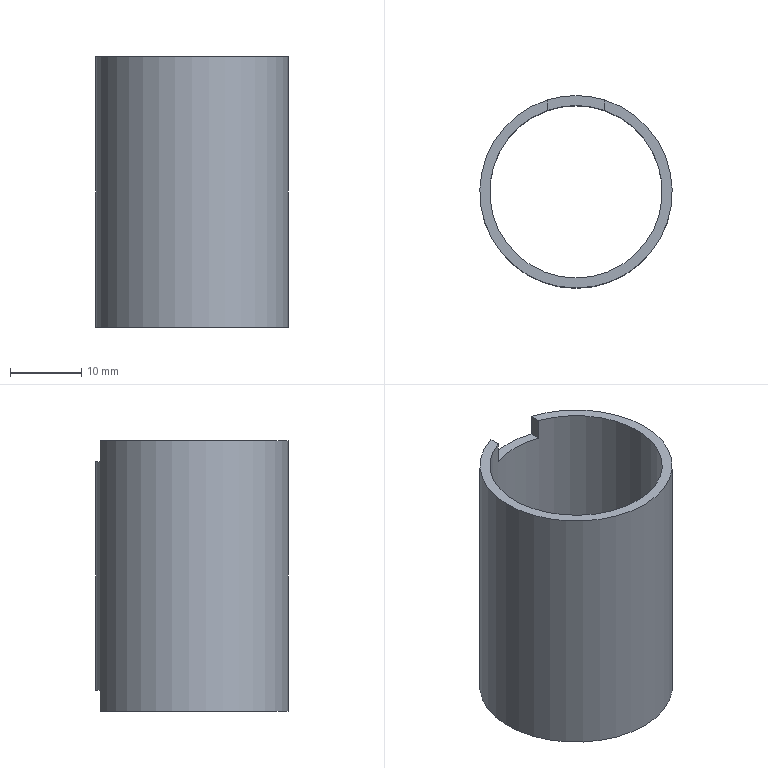Component | NX | UPPER_PISTON_CYLINDER_LINER | 1 solid | 10 faces | box 27 x 27 x 38 mm | volume 4210 mm3 | plane 8 | cylinder 2 | commonest cylinder face diameters 27 x1 24.2 x1
STEP:
#1=CARTESIAN_POINT('',(0.,0.,0.));
#2=DIRECTION('',(0.,0.,1.));
#3=DIRECTION('',(1.,0.,0.));
#4=AXIS2_PLACEMENT_3D('',#1,#2,#3);
#5=CARTESIAN_POINT('',(4.,2.894,162.5));
#6=VERTEX_POINT('',#5);
#7=CARTESIAN_POINT('',(4.,2.894,159.5));
#8=VERTEX_POINT('',#7);
#9=CARTESIAN_POINT('',(4.,2.894,162.5));
#10=DIRECTION('',(0.,0.,-1.));
#11=VECTOR('',#10,1.);
#12=LINE('',#9,#11);
#13=CARTESIAN_POINT('',(-0.,-10.,162.5));
#14=DIRECTION('',(0.,0.,-1.));
#15=DIRECTION('',(1.,0.,0.));
#16=AXIS2_PLACEMENT_3D('',#13,#14,#15);
#17=CYLINDRICAL_SURFACE('',#16,13.5);
#18=CARTESIAN_POINT('',(5.013,0.));
#19=DIRECTION('',(0.,1.));
#20=VECTOR('',#19,1.);
#21=LINE('',#18,#20);
#22=(GEOMETRIC_REPRESENTATION_CONTEXT(2)PARAMETRIC_REPRESENTATION_CONTEXT()REPRESENTATION_CONTEXT('',''));
#23=DEFINITIONAL_REPRESENTATION('',(#21),#22);
#24=PCURVE('',#17,#23);
#25=CARTESIAN_POINT('',(4.,-3.333,159.5));
#26=DIRECTION('',(1.,0.,0.));
#27=DIRECTION('',(0.,0.,1.));
#28=AXIS2_PLACEMENT_3D('',#25,#26,#27);
#29=PLANE('',#28);
#30=CARTESIAN_POINT('',(3.,-6.227));
#31=DIRECTION('',(-1.,0.));
#32=VECTOR('',#31,1.);
#33=LINE('',#30,#32);
#34=(GEOMETRIC_REPRESENTATION_CONTEXT(2)PARAMETRIC_REPRESENTATION_CONTEXT()REPRESENTATION_CONTEXT('',''));
#35=DEFINITIONAL_REPRESENTATION('',(#33),#34);
#36=PCURVE('',#29,#35);
#37=SURFACE_CURVE('',#12,(#24,#36),.PCURVE_S1.);
#38=EDGE_CURVE('',#6,#8,#37,.T.);
#39=ORIENTED_EDGE('',*,*,#38,.F.);
#40=CARTESIAN_POINT('',(-4.,2.894,162.5));
#41=VERTEX_POINT('',#40);
#42=CARTESIAN_POINT('',(-0.,-10.,162.5));
#43=DIRECTION('',(0.,0.,-1.));
#44=DIRECTION('',(-1.,-0.,0.));
#45=AXIS2_PLACEMENT_3D('',#42,#43,#44);
#46=CIRCLE('',#45,13.5);
#47=CARTESIAN_POINT('',(3.142,0.));
#48=DIRECTION('',(1.,0.));
#49=VECTOR('',#48,1.);
#50=LINE('',#47,#49);
#51=(GEOMETRIC_REPRESENTATION_CONTEXT(2)PARAMETRIC_REPRESENTATION_CONTEXT()REPRESENTATION_CONTEXT('',''));
#52=DEFINITIONAL_REPRESENTATION('',(#50),#51);
#53=PCURVE('',#17,#52);
#54=CARTESIAN_POINT('',(-0.,-10.,162.5));
#55=DIRECTION('',(0.,0.,-1.));
#56=DIRECTION('',(1.,0.,0.));
#57=AXIS2_PLACEMENT_3D('',#54,#55,#56);
#58=PLANE('',#57);
#59=CARTESIAN_POINT('',(0.,0.));
#60=DIRECTION('',(-1.,0.));
#61=AXIS2_PLACEMENT_2D('',#59,#60);
#62=CIRCLE('',#61,13.5);
#63=(GEOMETRIC_REPRESENTATION_CONTEXT(2)PARAMETRIC_REPRESENTATION_CONTEXT()REPRESENTATION_CONTEXT('',''));
#64=DEFINITIONAL_REPRESENTATION('',(#62),#63);
#65=PCURVE('',#58,#64);
#66=SURFACE_CURVE('',#46,(#53,#65),.PCURVE_S1.);
#67=EDGE_CURVE('',#6,#41,#66,.T.);
#68=ORIENTED_EDGE('',*,*,#67,.T.);
#69=CARTESIAN_POINT('',(-4.,2.894,159.5));
#70=VERTEX_POINT('',#69);
#71=CARTESIAN_POINT('',(-4.,2.894,162.5));
#72=DIRECTION('',(0.,0.,1.));
#73=VECTOR('',#72,1.);
#74=LINE('',#71,#73);
#75=CARTESIAN_POINT('',(10.695,0.));
#76=DIRECTION('',(0.,-1.));
#77=VECTOR('',#76,1.);
#78=LINE('',#75,#77);
#79=(GEOMETRIC_REPRESENTATION_CONTEXT(2)PARAMETRIC_REPRESENTATION_CONTEXT()REPRESENTATION_CONTEXT('',''));
#80=DEFINITIONAL_REPRESENTATION('',(#78),#79);
#81=PCURVE('',#17,#80);
#82=CARTESIAN_POINT('',(-4.,5.111,159.5));
#83=DIRECTION('',(-1.,0.,0.));
#84=DIRECTION('',(-0.,-1.,0.));
#85=AXIS2_PLACEMENT_3D('',#82,#83,#84);
#86=PLANE('',#85);
#87=CARTESIAN_POINT('',(2.217,3.));
#88=DIRECTION('',(0.,1.));
#89=VECTOR('',#88,1.);
#90=LINE('',#87,#89);
#91=(GEOMETRIC_REPRESENTATION_CONTEXT(2)PARAMETRIC_REPRESENTATION_CONTEXT()REPRESENTATION_CONTEXT('',''));
#92=DEFINITIONAL_REPRESENTATION('',(#90),#91);
#93=PCURVE('',#86,#92);
#94=SURFACE_CURVE('',#74,(#81,#93),.PCURVE_S1.);
#95=EDGE_CURVE('',#70,#41,#94,.T.);
#96=ORIENTED_EDGE('',*,*,#95,.F.);
#97=CARTESIAN_POINT('',(-0.,-10.,159.5));
#98=DIRECTION('',(0.,0.,-1.));
#99=DIRECTION('',(-1.,0.,0.));
#100=AXIS2_PLACEMENT_3D('',#97,#98,#99);
#101=CIRCLE('',#100,13.5);
#102=CARTESIAN_POINT('',(9.425,3.));
#103=DIRECTION('',(1.,0.));
#104=VECTOR('',#103,1.);
#105=LINE('',#102,#104);
#106=(GEOMETRIC_REPRESENTATION_CONTEXT(2)PARAMETRIC_REPRESENTATION_CONTEXT()REPRESENTATION_CONTEXT('',''));
#107=DEFINITIONAL_REPRESENTATION('',(#105),#106);
#108=PCURVE('',#17,#107);
#109=CARTESIAN_POINT('',(-0.,-10.,159.5));
#110=DIRECTION('',(0.,0.,1.));
#111=DIRECTION('',(-1.,0.,0.));
#112=AXIS2_PLACEMENT_3D('',#109,#110,#111);
#113=PLANE('',#112);
#114=CARTESIAN_POINT('',(13.5,0.));
#115=CARTESIAN_POINT('',(13.5,-23.383));
#116=CARTESIAN_POINT('',(-6.75,-11.691));
#117=CARTESIAN_POINT('',(-27.,-0.));
#118=CARTESIAN_POINT('',(-6.75,11.691));
#119=CARTESIAN_POINT('',(13.5,23.383));
#120=CARTESIAN_POINT('',(13.5,0.));
#121=(BOUNDED_CURVE()B_SPLINE_CURVE(2,(#114,#115,#116,#117,#118,#119,#120),.UNSPECIFIED.,.T.,.F.)B_SPLINE_CURVE_WITH_KNOTS((1,2,2,2,2,1),(-2.094,0.,2.094,4.189,6.283,8.378),.UNSPECIFIED.)CURVE()GEOMETRIC_REPRESENTATION_ITEM()RATIONAL_B_SPLINE_CURVE((1.,0.5,1.,0.5,1.,0.5,1.))REPRESENTATION_ITEM(''));
#122=(GEOMETRIC_REPRESENTATION_CONTEXT(2)PARAMETRIC_REPRESENTATION_CONTEXT()REPRESENTATION_CONTEXT('',''));
#123=DEFINITIONAL_REPRESENTATION('',(#121),#122);
#124=PCURVE('',#113,#123);
#125=SURFACE_CURVE('',#101,(#108,#124),.PCURVE_S1.);
#126=EDGE_CURVE('',#70,#8,#125,.T.);
#127=ORIENTED_EDGE('',*,*,#126,.T.);
#128=CARTESIAN_POINT('',(4.,2.894,127.5));
#129=VERTEX_POINT('',#128);
#130=CARTESIAN_POINT('',(4.,2.894,159.5));
#131=CARTESIAN_POINT('',(4.,2.894,127.5));
#132=B_SPLINE_CURVE_WITH_KNOTS('',1,(#130,#131),.UNSPECIFIED.,.F.,.F.,(2,2),(3.,35.),.PIECEWISE_BEZIER_KNOTS.);
#133=CARTESIAN_POINT('',(11.296,0.));
#134=DIRECTION('',(0.,1.));
#135=VECTOR('',#134,1.);
#136=LINE('',#133,#135);
#137=(GEOMETRIC_REPRESENTATION_CONTEXT(2)PARAMETRIC_REPRESENTATION_CONTEXT()REPRESENTATION_CONTEXT('',''));
#138=DEFINITIONAL_REPRESENTATION('',(#136),#137);
#139=PCURVE('',#17,#138);
#140=CARTESIAN_POINT('',(5.013,0.));
#141=DIRECTION('',(0.,1.));
#142=VECTOR('',#141,1.);
#143=LINE('',#140,#142);
#144=(GEOMETRIC_REPRESENTATION_CONTEXT(2)PARAMETRIC_REPRESENTATION_CONTEXT()REPRESENTATION_CONTEXT('',''));
#145=DEFINITIONAL_REPRESENTATION('',(#143),#144);
#146=PCURVE('',#17,#145);
#147=SEAM_CURVE('',#132,(#139,#146),.PCURVE_S1.);
#148=EDGE_CURVE('',#8,#129,#147,.T.);
#149=ORIENTED_EDGE('',*,*,#148,.T.);
#150=CARTESIAN_POINT('',(-4.,2.894,127.5));
#151=VERTEX_POINT('',#150);
#152=CARTESIAN_POINT('',(-0.,-10.,127.5));
#153=DIRECTION('',(0.,0.,-1.));
#154=DIRECTION('',(-1.,0.,0.));
#155=AXIS2_PLACEMENT_3D('',#152,#153,#154);
#156=CIRCLE('',#155,13.5);
#157=CARTESIAN_POINT('',(9.425,35.));
#158=DIRECTION('',(1.,0.));
#159=VECTOR('',#158,1.);
#160=LINE('',#157,#159);
#161=(GEOMETRIC_REPRESENTATION_CONTEXT(2)PARAMETRIC_REPRESENTATION_CONTEXT()REPRESENTATION_CONTEXT('',''));
#162=DEFINITIONAL_REPRESENTATION('',(#160),#161);
#163=PCURVE('',#17,#162);
#164=CARTESIAN_POINT('',(-0.,-10.,127.5));
#165=DIRECTION('',(0.,0.,1.));
#166=DIRECTION('',(-1.,0.,0.));
#167=AXIS2_PLACEMENT_3D('',#164,#165,#166);
#168=PLANE('',#167);
#169=CARTESIAN_POINT('',(13.5,0.));
#170=CARTESIAN_POINT('',(13.5,-23.383));
#171=CARTESIAN_POINT('',(-6.75,-11.691));
#172=CARTESIAN_POINT('',(-27.,-0.));
#173=CARTESIAN_POINT('',(-6.75,11.691));
#174=CARTESIAN_POINT('',(13.5,23.383));
#175=CARTESIAN_POINT('',(13.5,0.));
#176=(BOUNDED_CURVE()B_SPLINE_CURVE(2,(#169,#170,#171,#172,#173,#174,#175),.UNSPECIFIED.,.T.,.F.)B_SPLINE_CURVE_WITH_KNOTS((1,2,2,2,2,1),(-2.094,0.,2.094,4.189,6.283,8.378),.UNSPECIFIED.)CURVE()GEOMETRIC_REPRESENTATION_ITEM()RATIONAL_B_SPLINE_CURVE((1.,0.5,1.,0.5,1.,0.5,1.))REPRESENTATION_ITEM(''));
#177=(GEOMETRIC_REPRESENTATION_CONTEXT(2)PARAMETRIC_REPRESENTATION_CONTEXT()REPRESENTATION_CONTEXT('',''));
#178=DEFINITIONAL_REPRESENTATION('',(#176),#177);
#179=PCURVE('',#168,#178);
#180=SURFACE_CURVE('',#156,(#163,#179),.PCURVE_S1.);
#181=EDGE_CURVE('',#151,#129,#180,.T.);
#182=ORIENTED_EDGE('',*,*,#181,.F.);
#183=CARTESIAN_POINT('',(-4.,2.894,124.5));
#184=VERTEX_POINT('',#183);
#185=CARTESIAN_POINT('',(-4.,2.894,162.5));
#186=DIRECTION('',(0.,0.,-1.));
#187=VECTOR('',#186,1.);
#188=LINE('',#185,#187);
#189=CARTESIAN_POINT('',(10.695,0.));
#190=DIRECTION('',(0.,1.));
#191=VECTOR('',#190,1.);
#192=LINE('',#189,#191);
#193=(GEOMETRIC_REPRESENTATION_CONTEXT(2)PARAMETRIC_REPRESENTATION_CONTEXT()REPRESENTATION_CONTEXT('',''));
#194=DEFINITIONAL_REPRESENTATION('',(#192),#193);
#195=PCURVE('',#17,#194);
#196=CARTESIAN_POINT('',(-4.,5.111,127.5));
#197=DIRECTION('',(1.,-0.,0.));
#198=DIRECTION('',(0.,1.,0.));
#199=AXIS2_PLACEMENT_3D('',#196,#197,#198);
#200=PLANE('',#199);
#201=CARTESIAN_POINT('',(-2.217,35.));
#202=DIRECTION('',(0.,-1.));
#203=VECTOR('',#202,1.);
#204=LINE('',#201,#203);
#205=(GEOMETRIC_REPRESENTATION_CONTEXT(2)PARAMETRIC_REPRESENTATION_CONTEXT()REPRESENTATION_CONTEXT('',''));
#206=DEFINITIONAL_REPRESENTATION('',(#204),#205);
#207=PCURVE('',#200,#206);
#208=SURFACE_CURVE('',#188,(#195,#207),.PCURVE_S1.);
#209=EDGE_CURVE('',#151,#184,#208,.T.);
#210=ORIENTED_EDGE('',*,*,#209,.T.);
#211=CARTESIAN_POINT('',(4.,2.894,124.5));
#212=VERTEX_POINT('',#211);
#213=CARTESIAN_POINT('',(-0.,-10.,124.5));
#214=DIRECTION('',(0.,0.,-1.));
#215=DIRECTION('',(-1.,-0.,0.));
#216=AXIS2_PLACEMENT_3D('',#213,#214,#215);
#217=CIRCLE('',#216,13.5);
#218=CARTESIAN_POINT('',(3.142,38.));
#219=DIRECTION('',(1.,0.));
#220=VECTOR('',#219,1.);
#221=LINE('',#218,#220);
#222=(GEOMETRIC_REPRESENTATION_CONTEXT(2)PARAMETRIC_REPRESENTATION_CONTEXT()REPRESENTATION_CONTEXT('',''));
#223=DEFINITIONAL_REPRESENTATION('',(#221),#222);
#224=PCURVE('',#17,#223);
#225=CARTESIAN_POINT('',(-0.,-10.,124.5));
#226=DIRECTION('',(0.,0.,-1.));
#227=DIRECTION('',(1.,0.,0.));
#228=AXIS2_PLACEMENT_3D('',#225,#226,#227);
#229=PLANE('',#228);
#230=CARTESIAN_POINT('',(0.,0.));
#231=DIRECTION('',(-1.,0.));
#232=AXIS2_PLACEMENT_2D('',#230,#231);
#233=CIRCLE('',#232,13.5);
#234=(GEOMETRIC_REPRESENTATION_CONTEXT(2)PARAMETRIC_REPRESENTATION_CONTEXT()REPRESENTATION_CONTEXT('',''));
#235=DEFINITIONAL_REPRESENTATION('',(#233),#234);
#236=PCURVE('',#229,#235);
#237=SURFACE_CURVE('',#217,(#224,#236),.PCURVE_S1.);
#238=EDGE_CURVE('',#212,#184,#237,.T.);
#239=ORIENTED_EDGE('',*,*,#238,.F.);
#240=CARTESIAN_POINT('',(4.,2.894,162.5));
#241=DIRECTION('',(0.,0.,1.));
#242=VECTOR('',#241,1.);
#243=LINE('',#240,#242);
#244=CARTESIAN_POINT('',(5.013,0.));
#245=DIRECTION('',(0.,-1.));
#246=VECTOR('',#245,1.);
#247=LINE('',#244,#246);
#248=(GEOMETRIC_REPRESENTATION_CONTEXT(2)PARAMETRIC_REPRESENTATION_CONTEXT()REPRESENTATION_CONTEXT('',''));
#249=DEFINITIONAL_REPRESENTATION('',(#247),#248);
#250=PCURVE('',#17,#249);
#251=CARTESIAN_POINT('',(4.,-3.333,127.5));
#252=DIRECTION('',(-1.,0.,0.));
#253=DIRECTION('',(0.,0.,-1.));
#254=AXIS2_PLACEMENT_3D('',#251,#252,#253);
#255=PLANE('',#254);
#256=CARTESIAN_POINT('',(-35.,-6.227));
#257=DIRECTION('',(-1.,0.));
#258=VECTOR('',#257,1.);
#259=LINE('',#256,#258);
#260=(GEOMETRIC_REPRESENTATION_CONTEXT(2)PARAMETRIC_REPRESENTATION_CONTEXT()REPRESENTATION_CONTEXT('',''));
#261=DEFINITIONAL_REPRESENTATION('',(#259),#260);
#262=PCURVE('',#255,#261);
#263=SURFACE_CURVE('',#243,(#250,#262),.PCURVE_S1.);
#264=EDGE_CURVE('',#212,#129,#263,.T.);
#265=ORIENTED_EDGE('',*,*,#264,.T.);
#266=ORIENTED_EDGE('',*,*,#148,.F.);
#267=EDGE_LOOP('',(#39,#68,#96,#127,#149,#182,#210,#239,#265,#266));
#268=FACE_BOUND('',#267,.T.);
#269=ADVANCED_FACE('',(#268),#17,.T.);
#270=CARTESIAN_POINT('',(4.,1.42,124.5));
#271=VERTEX_POINT('',#270);
#272=CARTESIAN_POINT('',(-4.,1.42,124.5));
#273=VERTEX_POINT('',#272);
#274=CARTESIAN_POINT('',(0.,-10.,124.5));
#275=DIRECTION('',(0.,0.,-1.));
#276=DIRECTION('',(1.,0.,0.));
#277=AXIS2_PLACEMENT_3D('',#274,#275,#276);
#278=CIRCLE('',#277,12.1);
#279=CARTESIAN_POINT('',(0.,0.));
#280=DIRECTION('',(1.,0.));
#281=AXIS2_PLACEMENT_2D('',#279,#280);
#282=CIRCLE('',#281,12.1);
#283=(GEOMETRIC_REPRESENTATION_CONTEXT(2)PARAMETRIC_REPRESENTATION_CONTEXT()REPRESENTATION_CONTEXT('',''));
#284=DEFINITIONAL_REPRESENTATION('',(#282),#283);
#285=PCURVE('',#229,#284);
#286=CARTESIAN_POINT('',(0.,-10.,124.4));
#287=DIRECTION('',(0.,0.,1.));
#288=DIRECTION('',(-1.,0.,0.));
#289=AXIS2_PLACEMENT_3D('',#286,#287,#288);
#290=CYLINDRICAL_SURFACE('',#289,12.1);
#291=CARTESIAN_POINT('',(15.708,0.1));
#292=DIRECTION('',(-1.,0.));
#293=VECTOR('',#292,1.);
#294=LINE('',#291,#293);
#295=(GEOMETRIC_REPRESENTATION_CONTEXT(2)PARAMETRIC_REPRESENTATION_CONTEXT()REPRESENTATION_CONTEXT('',''));
#296=DEFINITIONAL_REPRESENTATION('',(#294),#295);
#297=PCURVE('',#290,#296);
#298=SURFACE_CURVE('',#278,(#285,#297),.PCURVE_S1.);
#299=EDGE_CURVE('',#271,#273,#298,.T.);
#300=ORIENTED_EDGE('',*,*,#299,.F.);
#301=CARTESIAN_POINT('',(4.,-3.333,124.5));
#302=DIRECTION('',(0.,1.,0.));
#303=VECTOR('',#302,1.);
#304=LINE('',#301,#303);
#305=CARTESIAN_POINT('',(4.,-6.667));
#306=DIRECTION('',(0.,-1.));
#307=VECTOR('',#306,1.);
#308=LINE('',#305,#307);
#309=(GEOMETRIC_REPRESENTATION_CONTEXT(2)PARAMETRIC_REPRESENTATION_CONTEXT()REPRESENTATION_CONTEXT('',''));
#310=DEFINITIONAL_REPRESENTATION('',(#308),#309);
#311=PCURVE('',#229,#310);
#312=CARTESIAN_POINT('',(3.,0.));
#313=DIRECTION('',(0.,-1.));
#314=VECTOR('',#313,1.);
#315=LINE('',#312,#314);
#316=(GEOMETRIC_REPRESENTATION_CONTEXT(2)PARAMETRIC_REPRESENTATION_CONTEXT()REPRESENTATION_CONTEXT('',''));
#317=DEFINITIONAL_REPRESENTATION('',(#315),#316);
#318=PCURVE('',#255,#317);
#319=SURFACE_CURVE('',#304,(#311,#318),.PCURVE_S1.);
#320=EDGE_CURVE('',#271,#212,#319,.T.);
#321=ORIENTED_EDGE('',*,*,#320,.T.);
#322=ORIENTED_EDGE('',*,*,#238,.T.);
#323=CARTESIAN_POINT('',(-4.,5.111,124.5));
#324=DIRECTION('',(-0.,-1.,0.));
#325=VECTOR('',#324,1.);
#326=LINE('',#323,#325);
#327=CARTESIAN_POINT('',(-4.,-15.111));
#328=DIRECTION('',(-0.,1.));
#329=VECTOR('',#328,1.);
#330=LINE('',#327,#329);
#331=(GEOMETRIC_REPRESENTATION_CONTEXT(2)PARAMETRIC_REPRESENTATION_CONTEXT()REPRESENTATION_CONTEXT('',''));
#332=DEFINITIONAL_REPRESENTATION('',(#330),#331);
#333=PCURVE('',#229,#332);
#334=CARTESIAN_POINT('',(0.,-3.));
#335=DIRECTION('',(-1.,0.));
#336=VECTOR('',#335,1.);
#337=LINE('',#334,#336);
#338=(GEOMETRIC_REPRESENTATION_CONTEXT(2)PARAMETRIC_REPRESENTATION_CONTEXT()REPRESENTATION_CONTEXT('',''));
#339=DEFINITIONAL_REPRESENTATION('',(#337),#338);
#340=PCURVE('',#200,#339);
#341=SURFACE_CURVE('',#326,(#333,#340),.PCURVE_S1.);
#342=EDGE_CURVE('',#184,#273,#341,.T.);
#343=ORIENTED_EDGE('',*,*,#342,.T.);
#344=EDGE_LOOP('',(#300,#321,#322,#343));
#345=FACE_BOUND('',#344,.T.);
#346=ADVANCED_FACE('',(#345),#229,.T.);
#347=CARTESIAN_POINT('',(4.,1.42,162.5));
#348=VERTEX_POINT('',#347);
#349=CARTESIAN_POINT('',(4.,-3.333,162.5));
#350=DIRECTION('',(0.,1.,0.));
#351=VECTOR('',#350,1.);
#352=LINE('',#349,#351);
#353=CARTESIAN_POINT('',(4.,-6.667));
#354=DIRECTION('',(0.,-1.));
#355=VECTOR('',#354,1.);
#356=LINE('',#353,#355);
#357=(GEOMETRIC_REPRESENTATION_CONTEXT(2)PARAMETRIC_REPRESENTATION_CONTEXT()REPRESENTATION_CONTEXT('',''));
#358=DEFINITIONAL_REPRESENTATION('',(#356),#357);
#359=PCURVE('',#58,#358);
#360=CARTESIAN_POINT('',(3.,0.));
#361=DIRECTION('',(0.,-1.));
#362=VECTOR('',#361,1.);
#363=LINE('',#360,#362);
#364=(GEOMETRIC_REPRESENTATION_CONTEXT(2)PARAMETRIC_REPRESENTATION_CONTEXT()REPRESENTATION_CONTEXT('',''));
#365=DEFINITIONAL_REPRESENTATION('',(#363),#364);
#366=PCURVE('',#29,#365);
#367=SURFACE_CURVE('',#352,(#359,#366),.PCURVE_S1.);
#368=EDGE_CURVE('',#348,#6,#367,.T.);
#369=ORIENTED_EDGE('',*,*,#368,.F.);
#370=CARTESIAN_POINT('',(-4.,1.42,162.5));
#371=VERTEX_POINT('',#370);
#372=CARTESIAN_POINT('',(0.,-10.,162.5));
#373=DIRECTION('',(0.,0.,-1.));
#374=DIRECTION('',(1.,0.,0.));
#375=AXIS2_PLACEMENT_3D('',#372,#373,#374);
#376=CIRCLE('',#375,12.1);
#377=CARTESIAN_POINT('',(0.,0.));
#378=DIRECTION('',(1.,0.));
#379=AXIS2_PLACEMENT_2D('',#377,#378);
#380=CIRCLE('',#379,12.1);
#381=(GEOMETRIC_REPRESENTATION_CONTEXT(2)PARAMETRIC_REPRESENTATION_CONTEXT()REPRESENTATION_CONTEXT('',''));
#382=DEFINITIONAL_REPRESENTATION('',(#380),#381);
#383=PCURVE('',#58,#382);
#384=CARTESIAN_POINT('',(15.708,38.1));
#385=DIRECTION('',(-1.,0.));
#386=VECTOR('',#385,1.);
#387=LINE('',#384,#386);
#388=(GEOMETRIC_REPRESENTATION_CONTEXT(2)PARAMETRIC_REPRESENTATION_CONTEXT()REPRESENTATION_CONTEXT('',''));
#389=DEFINITIONAL_REPRESENTATION('',(#387),#388);
#390=PCURVE('',#290,#389);
#391=SURFACE_CURVE('',#376,(#383,#390),.PCURVE_S1.);
#392=EDGE_CURVE('',#348,#371,#391,.T.);
#393=ORIENTED_EDGE('',*,*,#392,.T.);
#394=CARTESIAN_POINT('',(-4.,5.111,162.5));
#395=DIRECTION('',(-0.,-1.,0.));
#396=VECTOR('',#395,1.);
#397=LINE('',#394,#396);
#398=CARTESIAN_POINT('',(-4.,-15.111));
#399=DIRECTION('',(-0.,1.));
#400=VECTOR('',#399,1.);
#401=LINE('',#398,#400);
#402=(GEOMETRIC_REPRESENTATION_CONTEXT(2)PARAMETRIC_REPRESENTATION_CONTEXT()REPRESENTATION_CONTEXT('',''));
#403=DEFINITIONAL_REPRESENTATION('',(#401),#402);
#404=PCURVE('',#58,#403);
#405=CARTESIAN_POINT('',(0.,3.));
#406=DIRECTION('',(1.,0.));
#407=VECTOR('',#406,1.);
#408=LINE('',#405,#407);
#409=(GEOMETRIC_REPRESENTATION_CONTEXT(2)PARAMETRIC_REPRESENTATION_CONTEXT()REPRESENTATION_CONTEXT('',''));
#410=DEFINITIONAL_REPRESENTATION('',(#408),#409);
#411=PCURVE('',#86,#410);
#412=SURFACE_CURVE('',#397,(#404,#411),.PCURVE_S1.);
#413=EDGE_CURVE('',#41,#371,#412,.T.);
#414=ORIENTED_EDGE('',*,*,#413,.F.);
#415=ORIENTED_EDGE('',*,*,#67,.F.);
#416=EDGE_LOOP('',(#369,#393,#414,#415));
#417=FACE_BOUND('',#416,.T.);
#418=ADVANCED_FACE('',(#417),#58,.F.);
#419=CARTESIAN_POINT('',(4.,1.42,159.5));
#420=VERTEX_POINT('',#419);
#421=CARTESIAN_POINT('',(-4.,1.42,159.5));
#422=VERTEX_POINT('',#421);
#423=CARTESIAN_POINT('',(0.,-10.,159.5));
#424=DIRECTION('',(0.,0.,1.));
#425=DIRECTION('',(-1.,0.,0.));
#426=AXIS2_PLACEMENT_3D('',#423,#424,#425);
#427=CIRCLE('',#426,12.1);
#428=CARTESIAN_POINT('',(-0.,0.));
#429=DIRECTION('',(1.,0.));
#430=AXIS2_PLACEMENT_2D('',#428,#429);
#431=CIRCLE('',#430,12.1);
#432=(GEOMETRIC_REPRESENTATION_CONTEXT(2)PARAMETRIC_REPRESENTATION_CONTEXT()REPRESENTATION_CONTEXT('',''));
#433=DEFINITIONAL_REPRESENTATION('',(#431),#432);
#434=PCURVE('',#113,#433);
#435=CARTESIAN_POINT('',(6.283,35.1));
#436=DIRECTION('',(1.,0.));
#437=VECTOR('',#436,1.);
#438=LINE('',#435,#437);
#439=(GEOMETRIC_REPRESENTATION_CONTEXT(2)PARAMETRIC_REPRESENTATION_CONTEXT()REPRESENTATION_CONTEXT('',''));
#440=DEFINITIONAL_REPRESENTATION('',(#438),#439);
#441=PCURVE('',#290,#440);
#442=SURFACE_CURVE('',#427,(#434,#441),.PCURVE_S1.);
#443=EDGE_CURVE('',#420,#422,#442,.T.);
#444=ORIENTED_EDGE('',*,*,#443,.F.);
#445=CARTESIAN_POINT('',(4.,-3.333,159.5));
#446=DIRECTION('',(0.,-1.,0.));
#447=VECTOR('',#446,1.);
#448=LINE('',#445,#447);
#449=CARTESIAN_POINT('',(-4.,-6.667));
#450=DIRECTION('',(0.,1.));
#451=VECTOR('',#450,1.);
#452=LINE('',#449,#451);
#453=(GEOMETRIC_REPRESENTATION_CONTEXT(2)PARAMETRIC_REPRESENTATION_CONTEXT()REPRESENTATION_CONTEXT('',''));
#454=DEFINITIONAL_REPRESENTATION('',(#452),#453);
#455=PCURVE('',#113,#454);
#456=CARTESIAN_POINT('',(0.,0.));
#457=DIRECTION('',(0.,1.));
#458=VECTOR('',#457,1.);
#459=LINE('',#456,#458);
#460=(GEOMETRIC_REPRESENTATION_CONTEXT(2)PARAMETRIC_REPRESENTATION_CONTEXT()REPRESENTATION_CONTEXT('',''));
#461=DEFINITIONAL_REPRESENTATION('',(#459),#460);
#462=PCURVE('',#29,#461);
#463=SURFACE_CURVE('',#448,(#455,#462),.PCURVE_S1.);
#464=EDGE_CURVE('',#8,#420,#463,.T.);
#465=ORIENTED_EDGE('',*,*,#464,.F.);
#466=ORIENTED_EDGE('',*,*,#126,.F.);
#467=CARTESIAN_POINT('',(-4.,5.111,159.5));
#468=DIRECTION('',(0.,1.,0.));
#469=VECTOR('',#468,1.);
#470=LINE('',#467,#469);
#471=CARTESIAN_POINT('',(4.,-15.111));
#472=DIRECTION('',(-0.,-1.));
#473=VECTOR('',#472,1.);
#474=LINE('',#471,#473);
#475=(GEOMETRIC_REPRESENTATION_CONTEXT(2)PARAMETRIC_REPRESENTATION_CONTEXT()REPRESENTATION_CONTEXT('',''));
#476=DEFINITIONAL_REPRESENTATION('',(#474),#475);
#477=PCURVE('',#113,#476);
#478=CARTESIAN_POINT('',(0.,0.));
#479=DIRECTION('',(-1.,0.));
#480=VECTOR('',#479,1.);
#481=LINE('',#478,#480);
#482=(GEOMETRIC_REPRESENTATION_CONTEXT(2)PARAMETRIC_REPRESENTATION_CONTEXT()REPRESENTATION_CONTEXT('',''));
#483=DEFINITIONAL_REPRESENTATION('',(#481),#482);
#484=PCURVE('',#86,#483);
#485=SURFACE_CURVE('',#470,(#477,#484),.PCURVE_S1.);
#486=EDGE_CURVE('',#422,#70,#485,.T.);
#487=ORIENTED_EDGE('',*,*,#486,.F.);
#488=EDGE_LOOP('',(#444,#465,#466,#487));
#489=FACE_BOUND('',#488,.T.);
#490=ADVANCED_FACE('',(#489),#113,.T.);
#491=ORIENTED_EDGE('',*,*,#464,.T.);
#492=CARTESIAN_POINT('',(4.,1.42,124.4));
#493=DIRECTION('',(0.,0.,1.));
#494=VECTOR('',#493,1.);
#495=LINE('',#492,#494);
#496=CARTESIAN_POINT('',(-35.1,-4.753));
#497=DIRECTION('',(1.,0.));
#498=VECTOR('',#497,1.);
#499=LINE('',#496,#498);
#500=(GEOMETRIC_REPRESENTATION_CONTEXT(2)PARAMETRIC_REPRESENTATION_CONTEXT()REPRESENTATION_CONTEXT('',''));
#501=DEFINITIONAL_REPRESENTATION('',(#499),#500);
#502=PCURVE('',#29,#501);
#503=CARTESIAN_POINT('',(10.659,0.));
#504=DIRECTION('',(0.,1.));
#505=VECTOR('',#504,1.);
#506=LINE('',#503,#505);
#507=(GEOMETRIC_REPRESENTATION_CONTEXT(2)PARAMETRIC_REPRESENTATION_CONTEXT()REPRESENTATION_CONTEXT('',''));
#508=DEFINITIONAL_REPRESENTATION('',(#506),#507);
#509=PCURVE('',#290,#508);
#510=SURFACE_CURVE('',#495,(#502,#509),.PCURVE_S1.);
#511=EDGE_CURVE('',#420,#348,#510,.T.);
#512=ORIENTED_EDGE('',*,*,#511,.T.);
#513=ORIENTED_EDGE('',*,*,#368,.T.);
#514=ORIENTED_EDGE('',*,*,#38,.T.);
#515=EDGE_LOOP('',(#491,#512,#513,#514));
#516=FACE_BOUND('',#515,.T.);
#517=ADVANCED_FACE('',(#516),#29,.F.);
#518=ORIENTED_EDGE('',*,*,#413,.T.);
#519=CARTESIAN_POINT('',(-4.,1.42,124.4));
#520=DIRECTION('',(0.,0.,-1.));
#521=VECTOR('',#520,1.);
#522=LINE('',#519,#521);
#523=CARTESIAN_POINT('',(3.691,-35.1));
#524=DIRECTION('',(0.,-1.));
#525=VECTOR('',#524,1.);
#526=LINE('',#523,#525);
#527=(GEOMETRIC_REPRESENTATION_CONTEXT(2)PARAMETRIC_REPRESENTATION_CONTEXT()REPRESENTATION_CONTEXT('',''));
#528=DEFINITIONAL_REPRESENTATION('',(#526),#527);
#529=PCURVE('',#86,#528);
#530=CARTESIAN_POINT('',(5.049,0.));
#531=DIRECTION('',(0.,-1.));
#532=VECTOR('',#531,1.);
#533=LINE('',#530,#532);
#534=(GEOMETRIC_REPRESENTATION_CONTEXT(2)PARAMETRIC_REPRESENTATION_CONTEXT()REPRESENTATION_CONTEXT('',''));
#535=DEFINITIONAL_REPRESENTATION('',(#533),#534);
#536=PCURVE('',#290,#535);
#537=SURFACE_CURVE('',#522,(#529,#536),.PCURVE_S1.);
#538=EDGE_CURVE('',#371,#422,#537,.T.);
#539=ORIENTED_EDGE('',*,*,#538,.T.);
#540=ORIENTED_EDGE('',*,*,#486,.T.);
#541=ORIENTED_EDGE('',*,*,#95,.T.);
#542=EDGE_LOOP('',(#518,#539,#540,#541));
#543=FACE_BOUND('',#542,.T.);
#544=ADVANCED_FACE('',(#543),#86,.F.);
#545=CARTESIAN_POINT('',(4.,1.42,127.5));
#546=VERTEX_POINT('',#545);
#547=CARTESIAN_POINT('',(4.,-3.333,127.5));
#548=DIRECTION('',(0.,-1.,0.));
#549=VECTOR('',#548,1.);
#550=LINE('',#547,#549);
#551=CARTESIAN_POINT('',(-4.,-6.667));
#552=DIRECTION('',(0.,1.));
#553=VECTOR('',#552,1.);
#554=LINE('',#551,#553);
#555=(GEOMETRIC_REPRESENTATION_CONTEXT(2)PARAMETRIC_REPRESENTATION_CONTEXT()REPRESENTATION_CONTEXT('',''));
#556=DEFINITIONAL_REPRESENTATION('',(#554),#555);
#557=PCURVE('',#168,#556);
#558=CARTESIAN_POINT('',(0.,0.));
#559=DIRECTION('',(0.,1.));
#560=VECTOR('',#559,1.);
#561=LINE('',#558,#560);
#562=(GEOMETRIC_REPRESENTATION_CONTEXT(2)PARAMETRIC_REPRESENTATION_CONTEXT()REPRESENTATION_CONTEXT('',''));
#563=DEFINITIONAL_REPRESENTATION('',(#561),#562);
#564=PCURVE('',#255,#563);
#565=SURFACE_CURVE('',#550,(#557,#564),.PCURVE_S1.);
#566=EDGE_CURVE('',#129,#546,#565,.T.);
#567=ORIENTED_EDGE('',*,*,#566,.T.);
#568=CARTESIAN_POINT('',(-4.,1.42,127.5));
#569=VERTEX_POINT('',#568);
#570=CARTESIAN_POINT('',(0.,-10.,127.5));
#571=DIRECTION('',(0.,0.,1.));
#572=DIRECTION('',(-1.,0.,0.));
#573=AXIS2_PLACEMENT_3D('',#570,#571,#572);
#574=CIRCLE('',#573,12.1);
#575=CARTESIAN_POINT('',(-0.,0.));
#576=DIRECTION('',(1.,0.));
#577=AXIS2_PLACEMENT_2D('',#575,#576);
#578=CIRCLE('',#577,12.1);
#579=(GEOMETRIC_REPRESENTATION_CONTEXT(2)PARAMETRIC_REPRESENTATION_CONTEXT()REPRESENTATION_CONTEXT('',''));
#580=DEFINITIONAL_REPRESENTATION('',(#578),#579);
#581=PCURVE('',#168,#580);
#582=CARTESIAN_POINT('',(6.283,3.1));
#583=DIRECTION('',(1.,0.));
#584=VECTOR('',#583,1.);
#585=LINE('',#582,#584);
#586=(GEOMETRIC_REPRESENTATION_CONTEXT(2)PARAMETRIC_REPRESENTATION_CONTEXT()REPRESENTATION_CONTEXT('',''));
#587=DEFINITIONAL_REPRESENTATION('',(#585),#586);
#588=PCURVE('',#290,#587);
#589=SURFACE_CURVE('',#574,(#581,#588),.PCURVE_S1.);
#590=EDGE_CURVE('',#546,#569,#589,.T.);
#591=ORIENTED_EDGE('',*,*,#590,.T.);
#592=CARTESIAN_POINT('',(-4.,5.111,127.5));
#593=DIRECTION('',(0.,1.,0.));
#594=VECTOR('',#593,1.);
#595=LINE('',#592,#594);
#596=CARTESIAN_POINT('',(4.,-15.111));
#597=DIRECTION('',(-0.,-1.));
#598=VECTOR('',#597,1.);
#599=LINE('',#596,#598);
#600=(GEOMETRIC_REPRESENTATION_CONTEXT(2)PARAMETRIC_REPRESENTATION_CONTEXT()REPRESENTATION_CONTEXT('',''));
#601=DEFINITIONAL_REPRESENTATION('',(#599),#600);
#602=PCURVE('',#168,#601);
#603=CARTESIAN_POINT('',(0.,0.));
#604=DIRECTION('',(1.,0.));
#605=VECTOR('',#604,1.);
#606=LINE('',#603,#605);
#607=(GEOMETRIC_REPRESENTATION_CONTEXT(2)PARAMETRIC_REPRESENTATION_CONTEXT()REPRESENTATION_CONTEXT('',''));
#608=DEFINITIONAL_REPRESENTATION('',(#606),#607);
#609=PCURVE('',#200,#608);
#610=SURFACE_CURVE('',#595,(#602,#609),.PCURVE_S1.);
#611=EDGE_CURVE('',#569,#151,#610,.T.);
#612=ORIENTED_EDGE('',*,*,#611,.T.);
#613=ORIENTED_EDGE('',*,*,#181,.T.);
#614=EDGE_LOOP('',(#567,#591,#612,#613));
#615=FACE_BOUND('',#614,.T.);
#616=ADVANCED_FACE('',(#615),#168,.F.);
#617=CARTESIAN_POINT('',(4.,1.42,124.4));
#618=DIRECTION('',(0.,0.,-1.));
#619=VECTOR('',#618,1.);
#620=LINE('',#617,#619);
#621=CARTESIAN_POINT('',(3.1,-4.753));
#622=DIRECTION('',(1.,0.));
#623=VECTOR('',#622,1.);
#624=LINE('',#621,#623);
#625=(GEOMETRIC_REPRESENTATION_CONTEXT(2)PARAMETRIC_REPRESENTATION_CONTEXT()REPRESENTATION_CONTEXT('',''));
#626=DEFINITIONAL_REPRESENTATION('',(#624),#625);
#627=PCURVE('',#255,#626);
#628=CARTESIAN_POINT('',(10.659,0.));
#629=DIRECTION('',(0.,-1.));
#630=VECTOR('',#629,1.);
#631=LINE('',#628,#630);
#632=(GEOMETRIC_REPRESENTATION_CONTEXT(2)PARAMETRIC_REPRESENTATION_CONTEXT()REPRESENTATION_CONTEXT('',''));
#633=DEFINITIONAL_REPRESENTATION('',(#631),#632);
#634=PCURVE('',#290,#633);
#635=SURFACE_CURVE('',#620,(#627,#634),.PCURVE_S1.);
#636=EDGE_CURVE('',#546,#271,#635,.T.);
#637=ORIENTED_EDGE('',*,*,#636,.F.);
#638=ORIENTED_EDGE('',*,*,#566,.F.);
#639=ORIENTED_EDGE('',*,*,#264,.F.);
#640=ORIENTED_EDGE('',*,*,#320,.F.);
#641=EDGE_LOOP('',(#637,#638,#639,#640));
#642=FACE_BOUND('',#641,.T.);
#643=ADVANCED_FACE('',(#642),#255,.T.);
#644=CARTESIAN_POINT('',(-4.,1.42,124.4));
#645=DIRECTION('',(0.,0.,1.));
#646=VECTOR('',#645,1.);
#647=LINE('',#644,#646);
#648=CARTESIAN_POINT('',(-3.691,-3.1));
#649=DIRECTION('',(0.,1.));
#650=VECTOR('',#649,1.);
#651=LINE('',#648,#650);
#652=(GEOMETRIC_REPRESENTATION_CONTEXT(2)PARAMETRIC_REPRESENTATION_CONTEXT()REPRESENTATION_CONTEXT('',''));
#653=DEFINITIONAL_REPRESENTATION('',(#651),#652);
#654=PCURVE('',#200,#653);
#655=CARTESIAN_POINT('',(5.049,0.));
#656=DIRECTION('',(0.,1.));
#657=VECTOR('',#656,1.);
#658=LINE('',#655,#657);
#659=(GEOMETRIC_REPRESENTATION_CONTEXT(2)PARAMETRIC_REPRESENTATION_CONTEXT()REPRESENTATION_CONTEXT('',''));
#660=DEFINITIONAL_REPRESENTATION('',(#658),#659);
#661=PCURVE('',#290,#660);
#662=SURFACE_CURVE('',#647,(#654,#661),.PCURVE_S1.);
#663=EDGE_CURVE('',#273,#569,#662,.T.);
#664=ORIENTED_EDGE('',*,*,#663,.F.);
#665=ORIENTED_EDGE('',*,*,#342,.F.);
#666=ORIENTED_EDGE('',*,*,#209,.F.);
#667=ORIENTED_EDGE('',*,*,#611,.F.);
#668=EDGE_LOOP('',(#664,#665,#666,#667));
#669=FACE_BOUND('',#668,.T.);
#670=ADVANCED_FACE('',(#669),#200,.T.);
#671=ORIENTED_EDGE('',*,*,#590,.T.);
#672=CARTESIAN_POINT('',(-4.,1.42,127.5));
#673=CARTESIAN_POINT('',(-4.,1.42,159.5));
#674=B_SPLINE_CURVE_WITH_KNOTS('',1,(#672,#673),.UNSPECIFIED.,.F.,.F.,(2,2),(3.1,35.1),.PIECEWISE_BEZIER_KNOTS.);
#675=CARTESIAN_POINT('',(11.332,0.));
#676=DIRECTION('',(0.,1.));
#677=VECTOR('',#676,1.);
#678=LINE('',#675,#677);
#679=(GEOMETRIC_REPRESENTATION_CONTEXT(2)PARAMETRIC_REPRESENTATION_CONTEXT()REPRESENTATION_CONTEXT('',''));
#680=DEFINITIONAL_REPRESENTATION('',(#678),#679);
#681=PCURVE('',#290,#680);
#682=CARTESIAN_POINT('',(5.049,0.));
#683=DIRECTION('',(0.,1.));
#684=VECTOR('',#683,1.);
#685=LINE('',#682,#684);
#686=(GEOMETRIC_REPRESENTATION_CONTEXT(2)PARAMETRIC_REPRESENTATION_CONTEXT()REPRESENTATION_CONTEXT('',''));
#687=DEFINITIONAL_REPRESENTATION('',(#685),#686);
#688=PCURVE('',#290,#687);
#689=SEAM_CURVE('',#674,(#681,#688),.PCURVE_S1.);
#690=EDGE_CURVE('',#569,#422,#689,.T.);
#691=ORIENTED_EDGE('',*,*,#690,.T.);
#692=ORIENTED_EDGE('',*,*,#443,.F.);
#693=ORIENTED_EDGE('',*,*,#511,.T.);
#694=ORIENTED_EDGE('',*,*,#392,.T.);
#695=ORIENTED_EDGE('',*,*,#538,.T.);
#696=ORIENTED_EDGE('',*,*,#690,.F.);
#697=ORIENTED_EDGE('',*,*,#663,.F.);
#698=ORIENTED_EDGE('',*,*,#299,.F.);
#699=ORIENTED_EDGE('',*,*,#636,.F.);
#700=EDGE_LOOP('',(#671,#691,#692,#693,#694,#695,#696,#697,#698,#699));
#701=FACE_BOUND('',#700,.F.);
#702=ADVANCED_FACE('',(#701),#290,.F.);
#703=CLOSED_SHELL('',(#269,#346,#418,#490,#517,#544,#616,#643,#670,#702));
#704=MANIFOLD_SOLID_BREP('',#703);
#705=(LENGTH_UNIT()NAMED_UNIT(*)SI_UNIT(.MILLI.,.METRE.));
#706=UNCERTAINTY_MEASURE_WITH_UNIT(LENGTH_MEASURE(0.000002),#705,'','');
#707=(NAMED_UNIT(*)PLANE_ANGLE_UNIT()SI_UNIT($,.RADIAN.));
#708=(NAMED_UNIT(*)SI_UNIT($,.STERADIAN.)SOLID_ANGLE_UNIT());
#709=(GEOMETRIC_REPRESENTATION_CONTEXT(3)GLOBAL_UNCERTAINTY_ASSIGNED_CONTEXT((#706))GLOBAL_UNIT_ASSIGNED_CONTEXT((#705,#707,#708))REPRESENTATION_CONTEXT('',''));
#710=ADVANCED_BREP_SHAPE_REPRESENTATION('',(#4,#704),#709);